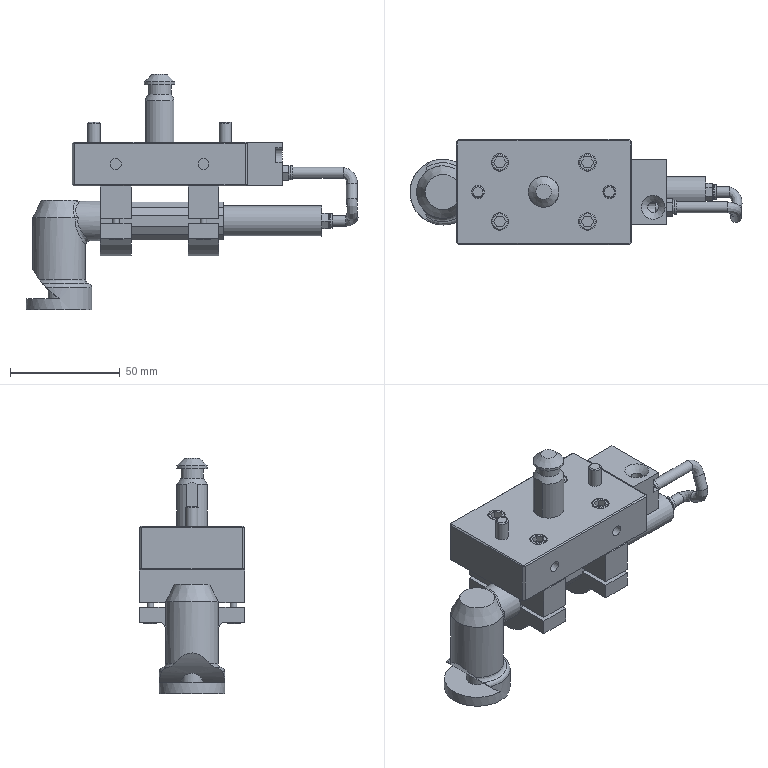Assembly | NX | mm | 21 component files | 22 solids | 379 faces | box 152.21 x 48 x 107.5 mm | volume 161813 mm3 | plane 229 | cylinder 90 | cone 45 | torus 8 | spline 4 | other 3 | commonest cylinder face diameters 5 x13 3.045 x8 6.5 x8 8 x8 3.3 x8 6 x7 4 x6 14 x5
Bill of materials:
unnamed part 1 | 4 |  | Revolved headed pin: short large-diameter cylindrical head with a long, smaller coaxial cylindrical shank; both ends have small chamfers.
unnamed part 2 | 1 |  | Round rod of constant diameter bent into several straight legs joined by radiused bends, with the legs lying in more than one plane.
unnamed part 3 | 2 |  | Plain solid cylinder with small edge breaks (fillets or chamfers) at both end faces.
unnamed part 4 | 2 |  | Saddle-shaped strap clamp: a central semicircular arch with a flat rectangular flange on each side, each flange having one vertical through-hole.
unnamed part 5 | 1 |  | Stepped revolved pin: a cone-topped flanged head, a reduced neck groove, a chamfered shoulder, a main cylindrical body and a smaller-diameter spigot at the bottom.
unnamed part 6 | 4 |  | Cap-screw-like part: cylindrical head with a hexagonal socket recess in the top, and a long, plain, smaller-diameter cylindrical shank with a chamfered tip.
unnamed part 7 | 2 |  | Hollow fitting-like body: a tapered round section on one side, a hexagonal flange in the middle, and a short cylindrical spigot with one circumferential groove on the other side; an axial bore runs through.
unnamed part 8 | 1 |  | Rectangular block with a countersunk through-hole on the top face, two round through-holes crossing the body, an open notch or slot at one end, and short cylindrical stubs sticking out from one side face.
unnamed part 9 | 1 |  | Rectangular plate or block with chamfered edges. The top face has a central counterbored through-hole, four through-holes in a rectangular pattern and two smaller blind holes. The side faces have blind drilled holes.
unnamed part 10 | 2 |  | Rectangular bar-shaped block with a semicircular cutout through its full width along the bottom face, and two holes in the top face.
unnamed part 11 | 1 |  | L-shaped revolved assembly-like body: a vertical cylindrical boss with a chamfered top and a larger base collar, joined at its side to a horizontal stepped round shaft that narrows toward a free end with a small axial hole.
Mates:
1. fix | robot_conn_plate 1 component
2. concentric | air_conn_block 1 arc | robot_conn_plate 1 edge
3. parallel | air_conn_block 1 face | robot_conn_plate 1 face
4. concentric | robot_conn_plate 1 edge | upper_conn_plate 2 edge
5. parallel | upper_conn_plate 2 face | robot_conn_plate 1 face
6. concentric | upper_conn_plate 1 edge | robot_conn_plate 1 edge
7. parallel | upper_conn_plate 1 face | upper_conn_plate 2 face
8. touch align | lower_fix_plate 2 face | upper_conn_plate 2 face
9. parallel | lower_fix_plate 2 face | upper_conn_plate 2 face
10. distance | lower_fix_plate 2 face | upper_conn_plate 2 face
11. touch align | lower_fix_plate 1 face | upper_conn_plate 1 face
12. parallel | lower_fix_plate 1 face | upper_conn_plate 1 face
13. distance | lower_fix_plate 1 face | upper_conn_plate 1 face
14. touch align | pneum_grinder_pen 1 face | lower_fix_plate 2 face
15. touch align | pneum_grinder_pen 1 face | lower_fix_plate 2 face
16. concentric | air_conn_block 1 edge | air_hose_conn 2 edge
17. parallel | air_hose_conn 2 face | air_conn_block 1 face
18. concentric | pneum_grinder_pen 1 arc | air_hose_conn 1 edge
19. concentric | hose 1 edge | air_hose_conn 2 edge
20. fix | hose 1 component
21. concentric | robot_conn_plate 1 edge | part 1 edge
22. concentric | part_2 2 edge | robot_conn_plate 1 edge
23. concentric | part_2 1 edge | robot_conn_plate 1 edge
24. concentric | screw 4 edge | robot_conn_plate 1 edge
25. concentric | screw 3 edge | robot_conn_plate 1 edge
26. concentric | screw 2 edge | robot_conn_plate 1 edge
27. concentric | screw 1 edge | robot_conn_plate 1 edge
28. concentric | screw_1 4 edge | lower_fix_plate 2 edge
29. concentric | screw_1 3 edge | lower_fix_plate 2 edge
30. concentric | screw_1 2 edge | lower_fix_plate 1 edge
31. concentric | screw_1 1 edge | lower_fix_plate 1 edge